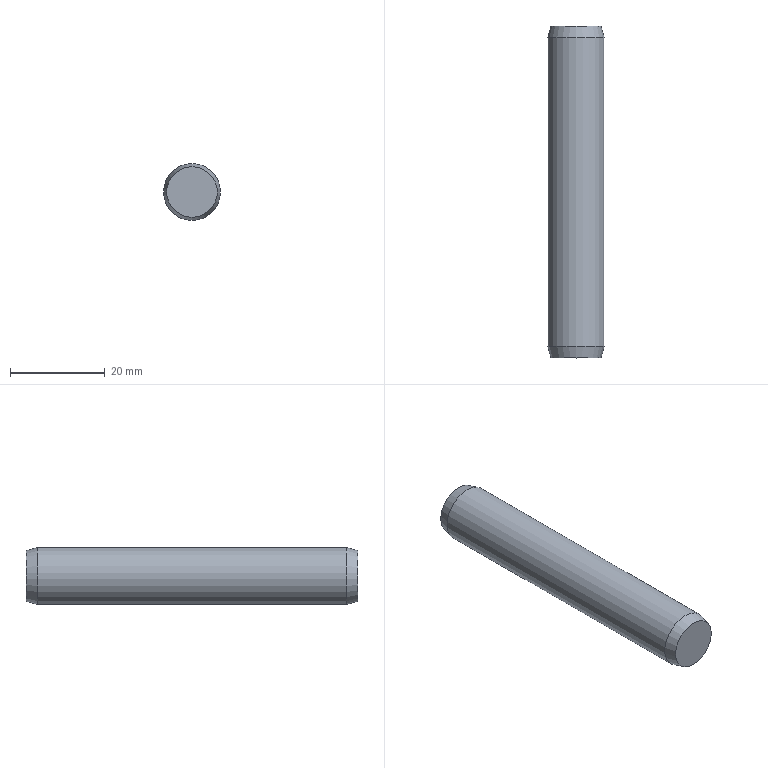Component | NX | GB-T119_1-2000_12X70 | 1 solid | 5 faces | box 12 x 70 x 12 mm | volume 7856 mm3 | plane 2 | cone 2 | cylinder 1 | commonest cylinder face diameters 12 x1
STEP:
#1=CARTESIAN_POINT('',(0.,0.,0.));
#2=DIRECTION('',(0.,0.,1.));
#3=DIRECTION('',(1.,0.,0.));
#4=AXIS2_PLACEMENT_3D('',#1,#2,#3);
#5=CARTESIAN_POINT('',(30.,12.,135.67));
#6=VERTEX_POINT('',#5);
#7=CARTESIAN_POINT('',(30.,12.,141.));
#8=DIRECTION('',(0.,1.,0.));
#9=DIRECTION('',(0.,0.,-1.));
#10=AXIS2_PLACEMENT_3D('',#7,#8,#9);
#11=CIRCLE('',#10,5.33);
#12=CARTESIAN_POINT('',(30.,12.,141.));
#13=DIRECTION('',(0.,1.,0.));
#14=DIRECTION('',(0.,0.,-1.));
#15=AXIS2_PLACEMENT_3D('',#12,#13,#14);
#16=PLANE('',#15);
#17=CARTESIAN_POINT('',(0.,0.));
#18=DIRECTION('',(1.,0.));
#19=AXIS2_PLACEMENT_2D('',#17,#18);
#20=CIRCLE('',#19,5.33);
#21=(GEOMETRIC_REPRESENTATION_CONTEXT(2)PARAMETRIC_REPRESENTATION_CONTEXT()REPRESENTATION_CONTEXT('',''));
#22=DEFINITIONAL_REPRESENTATION('',(#20),#21);
#23=PCURVE('',#16,#22);
#24=CARTESIAN_POINT('',(30.,12.,141.));
#25=DIRECTION('',(0.,-1.,0.));
#26=DIRECTION('',(0.,0.,1.));
#27=AXIS2_PLACEMENT_3D('',#24,#25,#26);
#28=CONICAL_SURFACE('',#27,5.33,0.2618);
#29=CARTESIAN_POINT('',(9.425,0.));
#30=DIRECTION('',(-1.,0.));
#31=VECTOR('',#30,1.);
#32=LINE('',#29,#31);
#33=(GEOMETRIC_REPRESENTATION_CONTEXT(2)PARAMETRIC_REPRESENTATION_CONTEXT()REPRESENTATION_CONTEXT('',''));
#34=DEFINITIONAL_REPRESENTATION('',(#32),#33);
#35=PCURVE('',#28,#34);
#36=SURFACE_CURVE('',#11,(#23,#35),.PCURVE_S1.);
#37=EDGE_CURVE('',#6,#6,#36,.T.);
#38=ORIENTED_EDGE('',*,*,#37,.T.);
#39=EDGE_LOOP('',(#38));
#40=FACE_BOUND('',#39,.T.);
#41=ADVANCED_FACE('',(#40),#16,.T.);
#42=CARTESIAN_POINT('',(30.,9.5,135.));
#43=VERTEX_POINT('',#42);
#44=CARTESIAN_POINT('',(30.,9.5,141.));
#45=DIRECTION('',(0.,1.,0.));
#46=DIRECTION('',(0.,0.,-1.));
#47=AXIS2_PLACEMENT_3D('',#44,#45,#46);
#48=CIRCLE('',#47,6.);
#49=CARTESIAN_POINT('',(9.425,2.5));
#50=DIRECTION('',(-1.,0.));
#51=VECTOR('',#50,1.);
#52=LINE('',#49,#51);
#53=(GEOMETRIC_REPRESENTATION_CONTEXT(2)PARAMETRIC_REPRESENTATION_CONTEXT()REPRESENTATION_CONTEXT('',''));
#54=DEFINITIONAL_REPRESENTATION('',(#52),#53);
#55=PCURVE('',#28,#54);
#56=CARTESIAN_POINT('',(30.,-58.,141.));
#57=DIRECTION('',(0.,1.,0.));
#58=DIRECTION('',(0.,0.,-1.));
#59=AXIS2_PLACEMENT_3D('',#56,#57,#58);
#60=CYLINDRICAL_SURFACE('',#59,6.);
#61=CARTESIAN_POINT('',(0.,67.5));
#62=DIRECTION('',(1.,0.));
#63=VECTOR('',#62,1.);
#64=LINE('',#61,#63);
#65=(GEOMETRIC_REPRESENTATION_CONTEXT(2)PARAMETRIC_REPRESENTATION_CONTEXT()REPRESENTATION_CONTEXT('',''));
#66=DEFINITIONAL_REPRESENTATION('',(#64),#65);
#67=PCURVE('',#60,#66);
#68=SURFACE_CURVE('',#48,(#55,#67),.PCURVE_S1.);
#69=EDGE_CURVE('',#43,#43,#68,.T.);
#70=ORIENTED_EDGE('',*,*,#69,.T.);
#71=CARTESIAN_POINT('',(30.,12.,135.67));
#72=CARTESIAN_POINT('',(30.,9.5,135.));
#73=B_SPLINE_CURVE_WITH_KNOTS('',1,(#71,#72),.UNSPECIFIED.,.F.,.F.,(2,2),(0.,2.588),.PIECEWISE_BEZIER_KNOTS.);
#74=CARTESIAN_POINT('',(3.142,0.));
#75=DIRECTION('',(0.,1.));
#76=VECTOR('',#75,1.);
#77=LINE('',#74,#76);
#78=(GEOMETRIC_REPRESENTATION_CONTEXT(2)PARAMETRIC_REPRESENTATION_CONTEXT()REPRESENTATION_CONTEXT('',''));
#79=DEFINITIONAL_REPRESENTATION('',(#77),#78);
#80=PCURVE('',#28,#79);
#81=CARTESIAN_POINT('',(9.425,0.));
#82=DIRECTION('',(0.,1.));
#83=VECTOR('',#82,1.);
#84=LINE('',#81,#83);
#85=(GEOMETRIC_REPRESENTATION_CONTEXT(2)PARAMETRIC_REPRESENTATION_CONTEXT()REPRESENTATION_CONTEXT('',''));
#86=DEFINITIONAL_REPRESENTATION('',(#84),#85);
#87=PCURVE('',#28,#86);
#88=SEAM_CURVE('',#73,(#80,#87),.PCURVE_S1.);
#89=EDGE_CURVE('',#6,#43,#88,.T.);
#90=ORIENTED_EDGE('',*,*,#89,.F.);
#91=ORIENTED_EDGE('',*,*,#37,.F.);
#92=ORIENTED_EDGE('',*,*,#89,.T.);
#93=EDGE_LOOP('',(#70,#90,#91,#92));
#94=FACE_BOUND('',#93,.T.);
#95=ADVANCED_FACE('',(#94),#28,.T.);
#96=CARTESIAN_POINT('',(30.,-55.5,135.));
#97=VERTEX_POINT('',#96);
#98=CARTESIAN_POINT('',(30.,-55.5,141.));
#99=DIRECTION('',(0.,1.,0.));
#100=DIRECTION('',(0.,0.,-1.));
#101=AXIS2_PLACEMENT_3D('',#98,#99,#100);
#102=CIRCLE('',#101,6.);
#103=CARTESIAN_POINT('',(0.,2.5));
#104=DIRECTION('',(1.,0.));
#105=VECTOR('',#104,1.);
#106=LINE('',#103,#105);
#107=(GEOMETRIC_REPRESENTATION_CONTEXT(2)PARAMETRIC_REPRESENTATION_CONTEXT()REPRESENTATION_CONTEXT('',''));
#108=DEFINITIONAL_REPRESENTATION('',(#106),#107);
#109=PCURVE('',#60,#108);
#110=CARTESIAN_POINT('',(30.,-55.5,141.));
#111=DIRECTION('',(0.,1.,0.));
#112=DIRECTION('',(0.,0.,-1.));
#113=AXIS2_PLACEMENT_3D('',#110,#111,#112);
#114=CONICAL_SURFACE('',#113,6.,0.2618);
#115=CARTESIAN_POINT('',(0.,0.));
#116=DIRECTION('',(1.,0.));
#117=VECTOR('',#116,1.);
#118=LINE('',#115,#117);
#119=(GEOMETRIC_REPRESENTATION_CONTEXT(2)PARAMETRIC_REPRESENTATION_CONTEXT()REPRESENTATION_CONTEXT('',''));
#120=DEFINITIONAL_REPRESENTATION('',(#118),#119);
#121=PCURVE('',#114,#120);
#122=SURFACE_CURVE('',#102,(#109,#121),.PCURVE_S1.);
#123=EDGE_CURVE('',#97,#97,#122,.T.);
#124=ORIENTED_EDGE('',*,*,#123,.T.);
#125=CARTESIAN_POINT('',(30.,-55.5,135.));
#126=CARTESIAN_POINT('',(30.,9.5,135.));
#127=B_SPLINE_CURVE_WITH_KNOTS('',1,(#125,#126),.UNSPECIFIED.,.F.,.F.,(2,2),(2.5,67.5),.PIECEWISE_BEZIER_KNOTS.);
#128=CARTESIAN_POINT('',(6.283,0.));
#129=DIRECTION('',(0.,1.));
#130=VECTOR('',#129,1.);
#131=LINE('',#128,#130);
#132=(GEOMETRIC_REPRESENTATION_CONTEXT(2)PARAMETRIC_REPRESENTATION_CONTEXT()REPRESENTATION_CONTEXT('',''));
#133=DEFINITIONAL_REPRESENTATION('',(#131),#132);
#134=PCURVE('',#60,#133);
#135=CARTESIAN_POINT('',(0.,0.));
#136=DIRECTION('',(0.,1.));
#137=VECTOR('',#136,1.);
#138=LINE('',#135,#137);
#139=(GEOMETRIC_REPRESENTATION_CONTEXT(2)PARAMETRIC_REPRESENTATION_CONTEXT()REPRESENTATION_CONTEXT('',''));
#140=DEFINITIONAL_REPRESENTATION('',(#138),#139);
#141=PCURVE('',#60,#140);
#142=SEAM_CURVE('',#127,(#134,#141),.PCURVE_S1.);
#143=EDGE_CURVE('',#97,#43,#142,.T.);
#144=ORIENTED_EDGE('',*,*,#143,.T.);
#145=ORIENTED_EDGE('',*,*,#69,.F.);
#146=ORIENTED_EDGE('',*,*,#143,.F.);
#147=EDGE_LOOP('',(#124,#144,#145,#146));
#148=FACE_BOUND('',#147,.T.);
#149=ADVANCED_FACE('',(#148),#60,.T.);
#150=CARTESIAN_POINT('',(30.,-58.,135.67));
#151=VERTEX_POINT('',#150);
#152=CARTESIAN_POINT('',(30.,-58.,141.));
#153=DIRECTION('',(0.,1.,0.));
#154=DIRECTION('',(0.,0.,-1.));
#155=AXIS2_PLACEMENT_3D('',#152,#153,#154);
#156=CIRCLE('',#155,5.33);
#157=CARTESIAN_POINT('',(0.,-2.5));
#158=DIRECTION('',(1.,0.));
#159=VECTOR('',#158,1.);
#160=LINE('',#157,#159);
#161=(GEOMETRIC_REPRESENTATION_CONTEXT(2)PARAMETRIC_REPRESENTATION_CONTEXT()REPRESENTATION_CONTEXT('',''));
#162=DEFINITIONAL_REPRESENTATION('',(#160),#161);
#163=PCURVE('',#114,#162);
#164=CARTESIAN_POINT('',(30.,-58.,146.33));
#165=DIRECTION('',(0.,-1.,0.));
#166=DIRECTION('',(0.,0.,1.));
#167=AXIS2_PLACEMENT_3D('',#164,#165,#166);
#168=PLANE('',#167);
#169=CARTESIAN_POINT('',(-10.66,0.));
#170=CARTESIAN_POINT('',(-10.66,9.232));
#171=CARTESIAN_POINT('',(-2.665,4.616));
#172=CARTESIAN_POINT('',(5.33,0.));
#173=CARTESIAN_POINT('',(-2.665,-4.616));
#174=CARTESIAN_POINT('',(-10.66,-9.232));
#175=CARTESIAN_POINT('',(-10.66,0.));
#176=(BOUNDED_CURVE()B_SPLINE_CURVE(2,(#169,#170,#171,#172,#173,#174,#175),.UNSPECIFIED.,.T.,.F.)B_SPLINE_CURVE_WITH_KNOTS((1,2,2,2,2,1),(-2.094,0.,2.094,4.189,6.283,8.378),.UNSPECIFIED.)CURVE()GEOMETRIC_REPRESENTATION_ITEM()RATIONAL_B_SPLINE_CURVE((1.,0.5,1.,0.5,1.,0.5,1.))REPRESENTATION_ITEM(''));
#177=(GEOMETRIC_REPRESENTATION_CONTEXT(2)PARAMETRIC_REPRESENTATION_CONTEXT()REPRESENTATION_CONTEXT('',''));
#178=DEFINITIONAL_REPRESENTATION('',(#176),#177);
#179=PCURVE('',#168,#178);
#180=SURFACE_CURVE('',#156,(#163,#179),.PCURVE_S1.);
#181=EDGE_CURVE('',#151,#151,#180,.T.);
#182=ORIENTED_EDGE('',*,*,#181,.T.);
#183=CARTESIAN_POINT('',(30.,-58.,135.67));
#184=CARTESIAN_POINT('',(30.,-55.5,135.));
#185=B_SPLINE_CURVE_WITH_KNOTS('',1,(#183,#184),.UNSPECIFIED.,.F.,.F.,(2,2),(-2.588,0.),.PIECEWISE_BEZIER_KNOTS.);
#186=CARTESIAN_POINT('',(6.283,0.));
#187=DIRECTION('',(0.,1.));
#188=VECTOR('',#187,1.);
#189=LINE('',#186,#188);
#190=(GEOMETRIC_REPRESENTATION_CONTEXT(2)PARAMETRIC_REPRESENTATION_CONTEXT()REPRESENTATION_CONTEXT('',''));
#191=DEFINITIONAL_REPRESENTATION('',(#189),#190);
#192=PCURVE('',#114,#191);
#193=CARTESIAN_POINT('',(0.,0.));
#194=DIRECTION('',(0.,1.));
#195=VECTOR('',#194,1.);
#196=LINE('',#193,#195);
#197=(GEOMETRIC_REPRESENTATION_CONTEXT(2)PARAMETRIC_REPRESENTATION_CONTEXT()REPRESENTATION_CONTEXT('',''));
#198=DEFINITIONAL_REPRESENTATION('',(#196),#197);
#199=PCURVE('',#114,#198);
#200=SEAM_CURVE('',#185,(#192,#199),.PCURVE_S1.);
#201=EDGE_CURVE('',#151,#97,#200,.T.);
#202=ORIENTED_EDGE('',*,*,#201,.T.);
#203=ORIENTED_EDGE('',*,*,#123,.F.);
#204=ORIENTED_EDGE('',*,*,#201,.F.);
#205=EDGE_LOOP('',(#182,#202,#203,#204));
#206=FACE_BOUND('',#205,.T.);
#207=ADVANCED_FACE('',(#206),#114,.T.);
#208=ORIENTED_EDGE('',*,*,#181,.F.);
#209=EDGE_LOOP('',(#208));
#210=FACE_BOUND('',#209,.T.);
#211=ADVANCED_FACE('',(#210),#168,.T.);
#212=CLOSED_SHELL('',(#41,#95,#149,#207,#211));
#213=MANIFOLD_SOLID_BREP('',#212);
#214=(LENGTH_UNIT()NAMED_UNIT(*)SI_UNIT(.MILLI.,.METRE.));
#215=UNCERTAINTY_MEASURE_WITH_UNIT(LENGTH_MEASURE(0.00001),#214,'','');
#216=(NAMED_UNIT(*)PLANE_ANGLE_UNIT()SI_UNIT($,.RADIAN.));
#217=(NAMED_UNIT(*)SI_UNIT($,.STERADIAN.)SOLID_ANGLE_UNIT());
#218=(GEOMETRIC_REPRESENTATION_CONTEXT(3)GLOBAL_UNCERTAINTY_ASSIGNED_CONTEXT((#215))GLOBAL_UNIT_ASSIGNED_CONTEXT((#214,#216,#217))REPRESENTATION_CONTEXT('',''));
#219=ADVANCED_BREP_SHAPE_REPRESENTATION('',(#4,#213),#218);